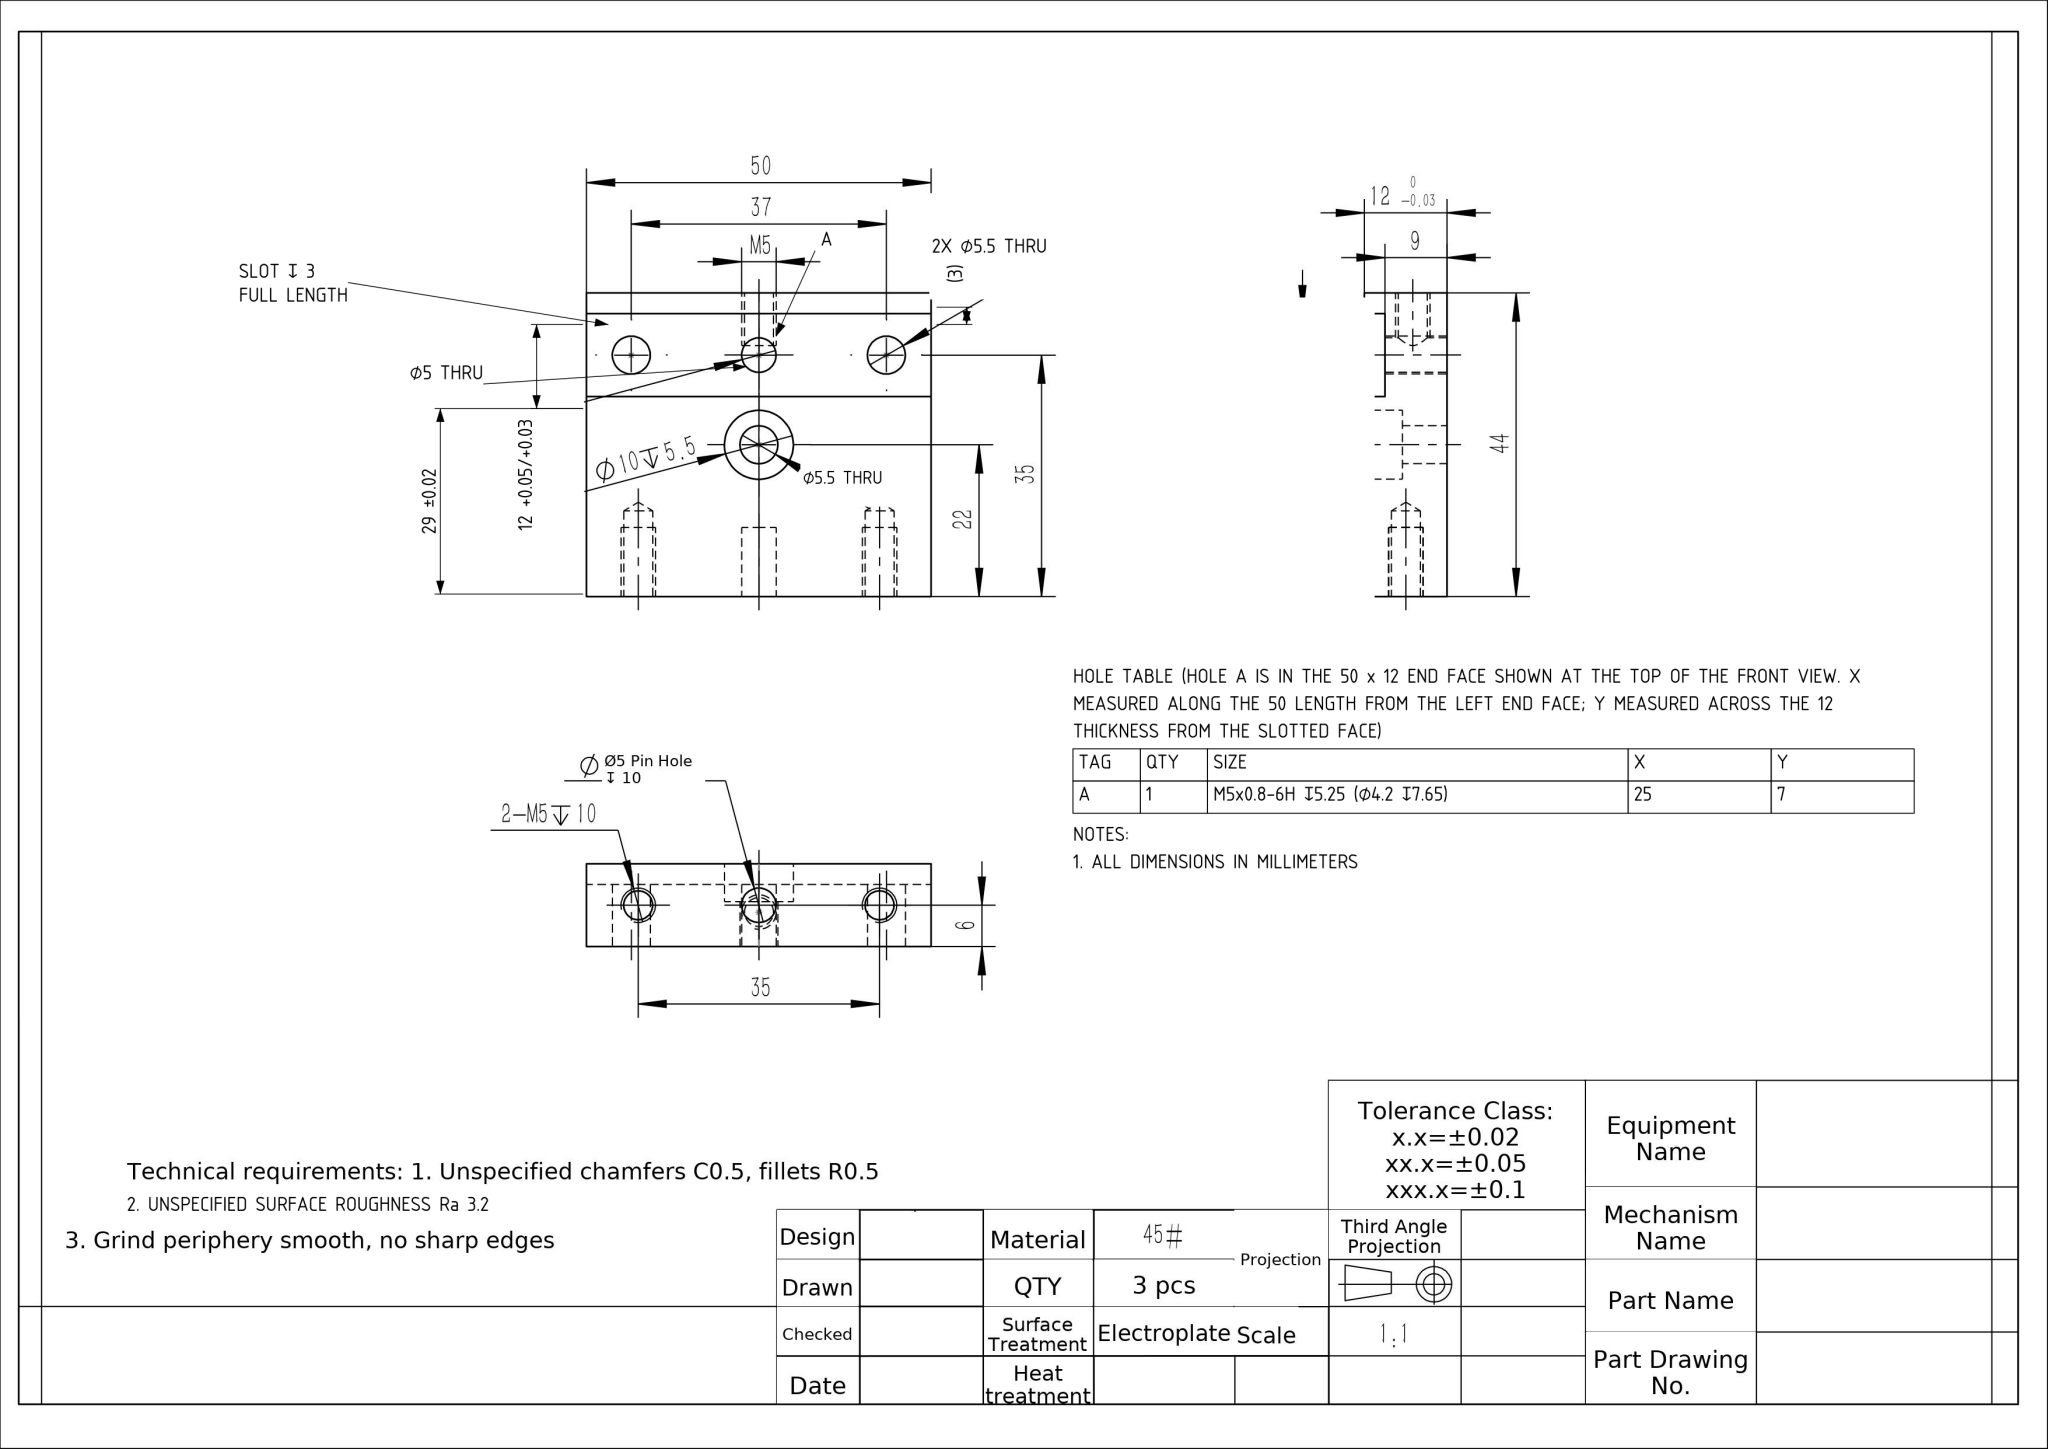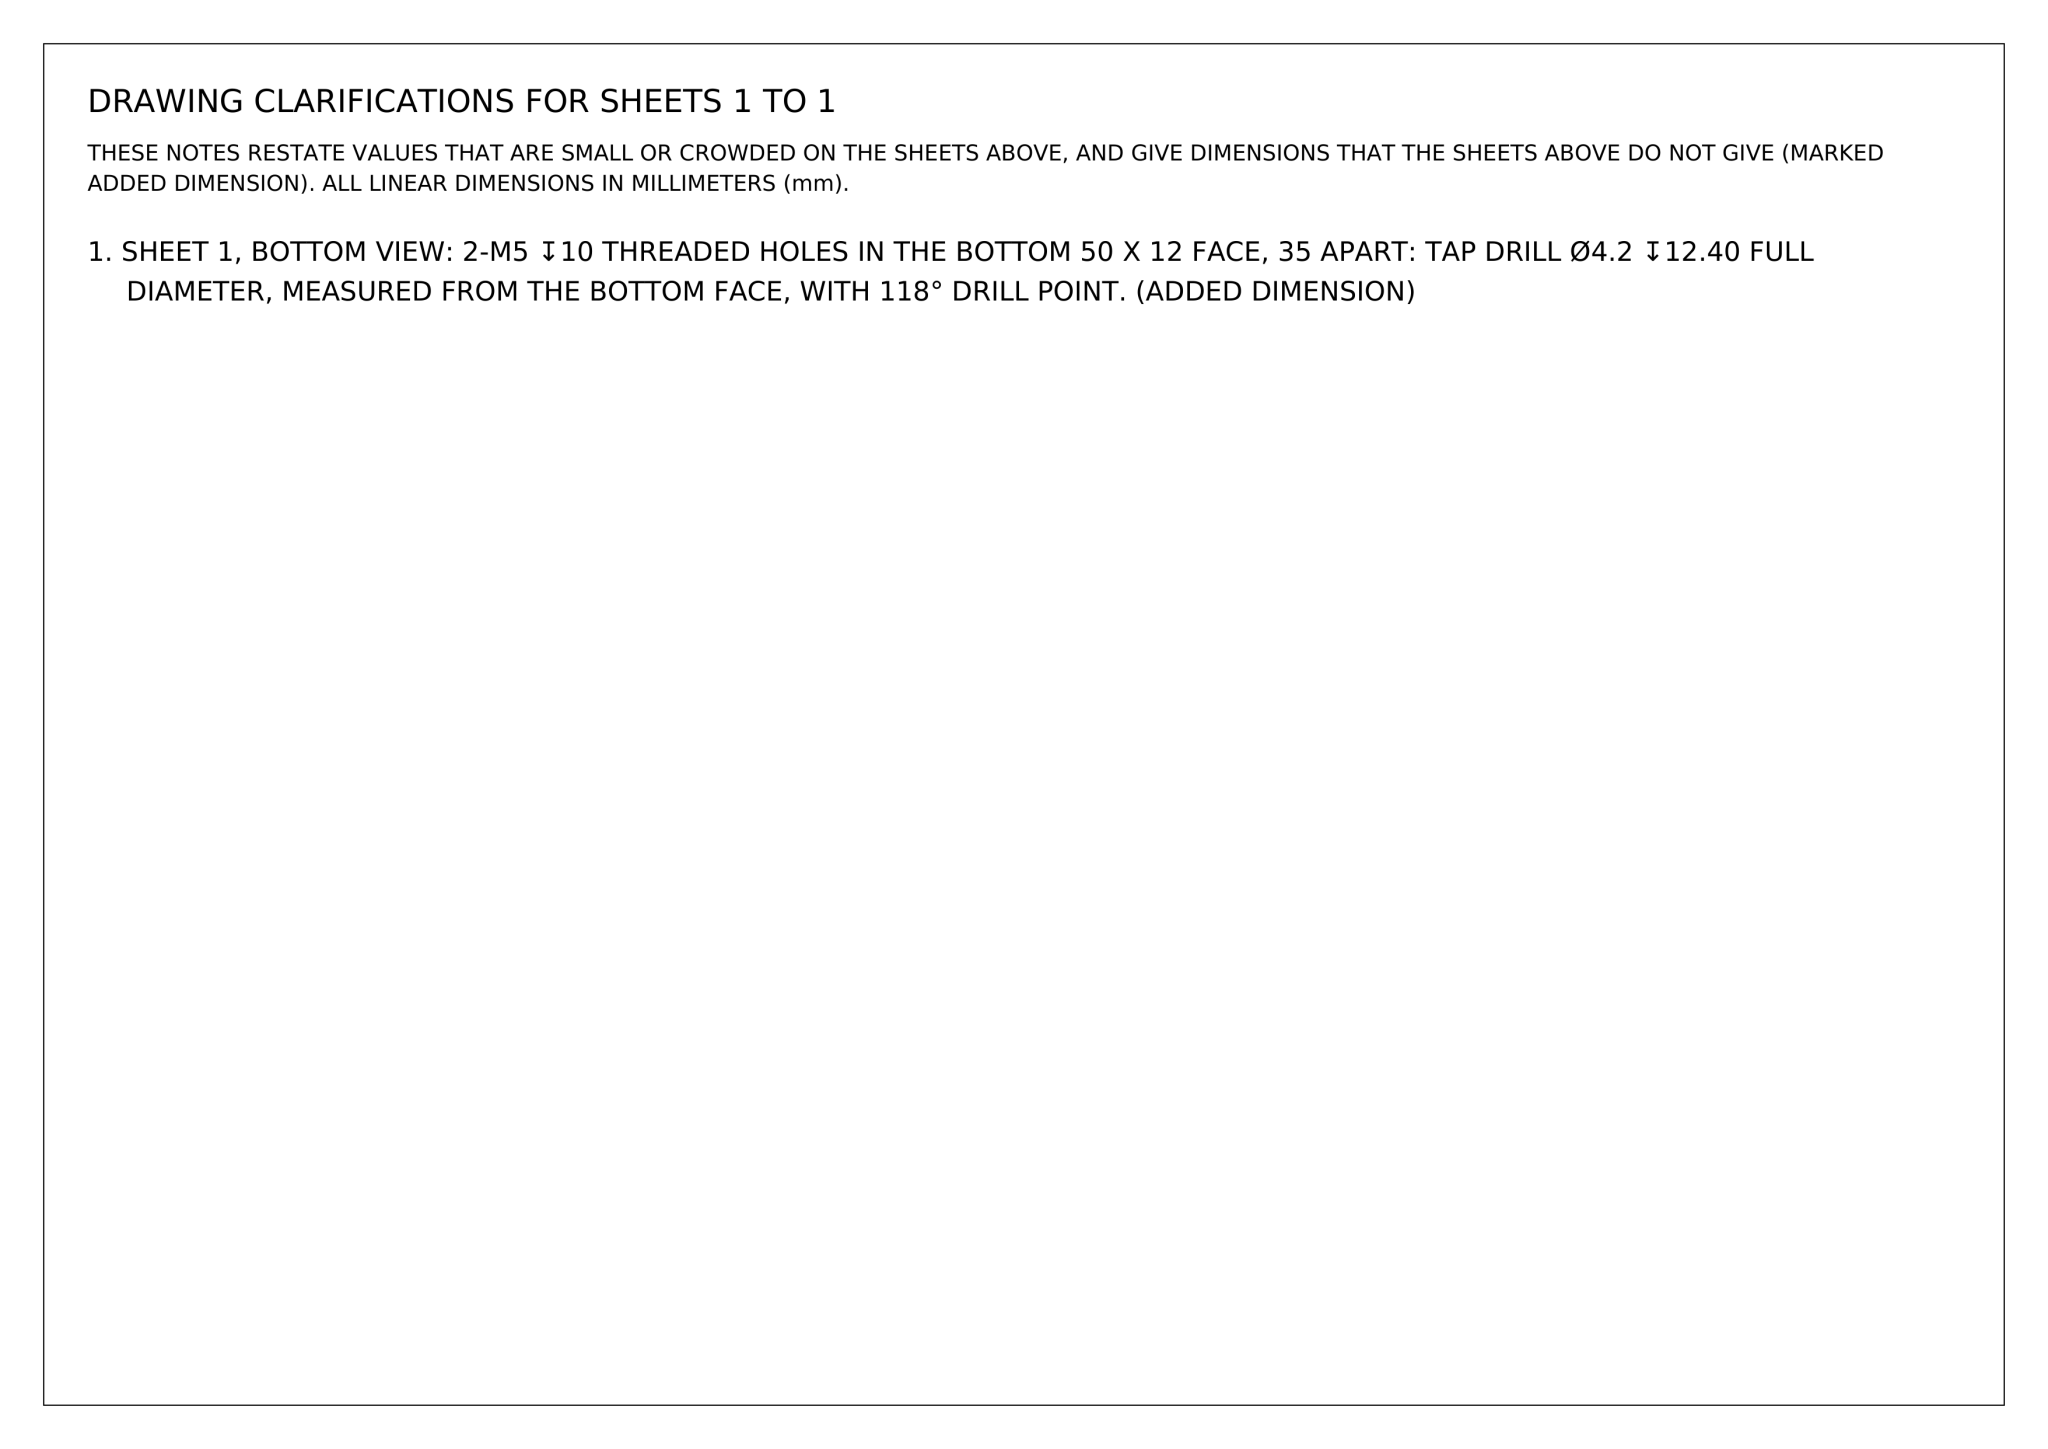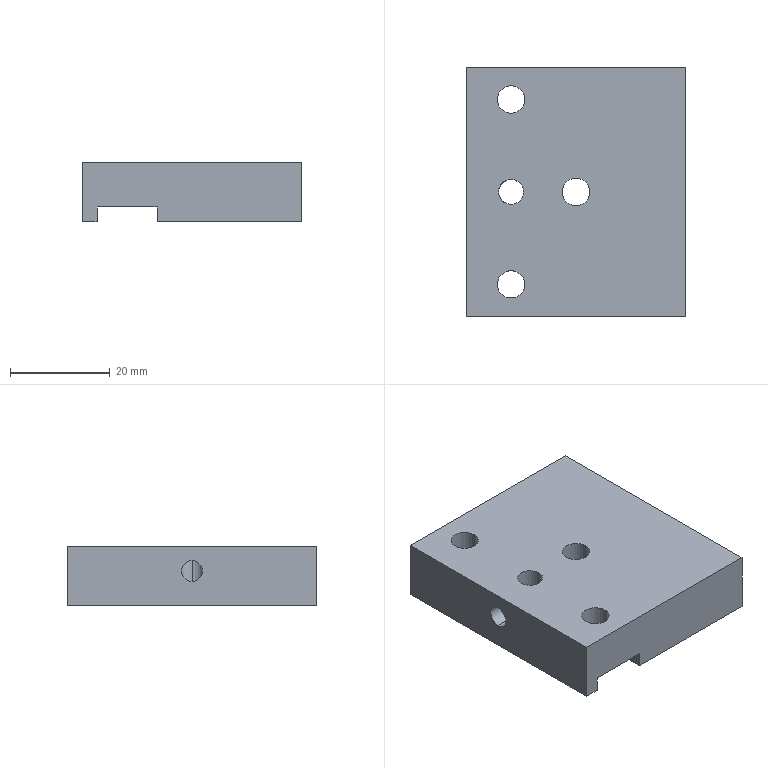Part | NX | mm | 1 solid | 34 faces | box 44 x 50 x 12 mm | volume 22764 mm3 | cylinder 18 | plane 12 | cone 4 | commonest cylinder face diameters 5.5 x6 4.2 x6 5 x4 10 x2